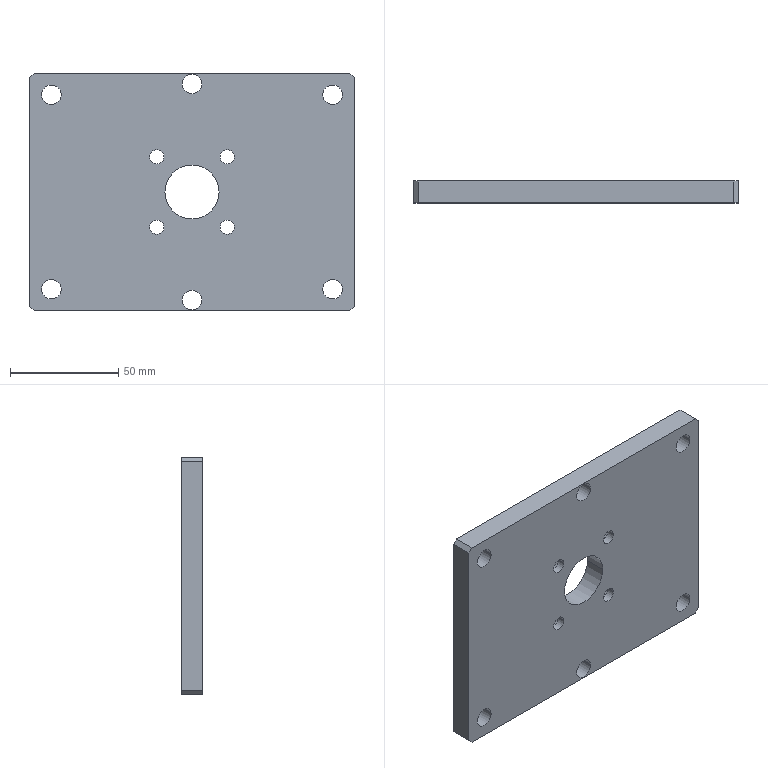Component | SolidWorks | 20-MaterialTrayLifting-1111-1_23-1111-2 | 1 solid | 56 faces | box 150 x 10 x 110 mm | volume 152169 mm3 | cylinder 38 | plane 18 | commonest cylinder face diameters 9 x12 11 x8 6.6 x8 16 x8 25 x2 | material A6061
build123d program:
from build123d import *

# Parameters (mm, degrees)
SKETCH1_W                                       = 150
SKETCH1_H                                       = 110
BOSS_EXTRUDE1_DEPTH                             = 10
SKETCH2_R                                       = 12.5
CUT_EXTRUDE1_DEPTH                              = 94.541
M8_CLEARANCE_HOLE_1_D                           = 9
SKETCH5_R                                       = 8
CUT_EXTRUDE2_DEPTH                              = 2
M10X1_0_TAPPED_HOLE1_D                          = 9
M6_HEX_SOCKET_HEAD_CAP_SCREW_CBORE1_D           = 6.6
M6_HEX_SOCKET_HEAD_CAP_SCREW_CBORE1_CBORE_D     = 11
M6_HEX_SOCKET_HEAD_CAP_SCREW_CBORE1_CBORE_DEPTH = 6.4
CHAMFER1_SIZE                                   = 2


with BuildPart() as part:
    # Sketch1 → Boss-Extrude1 (new body)
    with BuildSketch(Plane.XY):
        Rectangle(SKETCH1_W, SKETCH1_H)
    extrude(amount=BOSS_EXTRUDE1_DEPTH)

    # Sketch2 → Cut-Extrude1 (cut, through all)
    with BuildSketch(Plane(origin=(0, 0, 0), x_dir=(-1, 0, 0), z_dir=(0, 0, -1))):
        Circle(SKETCH2_R)
    extrude(amount=-CUT_EXTRUDE1_DEPTH, mode=Mode.SUBTRACT)

    # M8 Clearance Hole 1 (through all)
    with Locations(Plane.XY.offset(10)):
        with Locations((65, -45), (-65, 45), (65, 45), (-65, -45)):
            Hole(M8_CLEARANCE_HOLE_1_D / 2)

    # Sketch5 → Cut-Extrude2 (cut)
    with BuildSketch(Plane(origin=(0, 0, 0), x_dir=(-1, 0, 0), z_dir=(0, 0, -1))):
        with Locations((-65, 45)):
            Circle(SKETCH5_R)
        with Locations((65, 45)):
            Circle(SKETCH5_R)
        with Locations((-65, -45)):
            Circle(SKETCH5_R)
        with Locations((65, -45)):
            Circle(SKETCH5_R)
    extrude(amount=-CUT_EXTRUDE2_DEPTH, mode=Mode.SUBTRACT)

    # M10x1.0 Tapped Hole1 (through all)
    with Locations(Plane(origin=(0, 0, 0), x_dir=(-1, 0, 0), z_dir=(0, 0, -1))):
        with Locations((0, 50), (0, -50)):
            Hole(M10X1_0_TAPPED_HOLE1_D / 2)

    # M6 Hex Socket Head Cap Screw CBORE1 (through all)
    with Locations(Plane(origin=(0, 0, 0), x_dir=(-1, 0, 0), z_dir=(0, 0, -1))):
        with Locations((16.25, 16.25), (16.25, -16.25), (-16.25, -16.25), (-16.25, 16.25)):
            CounterBoreHole(M6_HEX_SOCKET_HEAD_CAP_SCREW_CBORE1_D / 2, M6_HEX_SOCKET_HEAD_CAP_SCREW_CBORE1_CBORE_D / 2, M6_HEX_SOCKET_HEAD_CAP_SCREW_CBORE1_CBORE_DEPTH)

    # Chamfer1
    chamfer1_edges = [part.edges().sort_by_distance(p)[0] for p in [
        (75, -55, 5),
        (-75, -55, 5),
        (-75, 55, 5),
        (75, 55, 5),
    ]]
    chamfer(chamfer1_edges, length=CHAMFER1_SIZE)


solid = part.part

# Placed as in the assembly
solid = solid.moved(Location((3.428, 291.224, 1393.056), (90, 0, 0)))